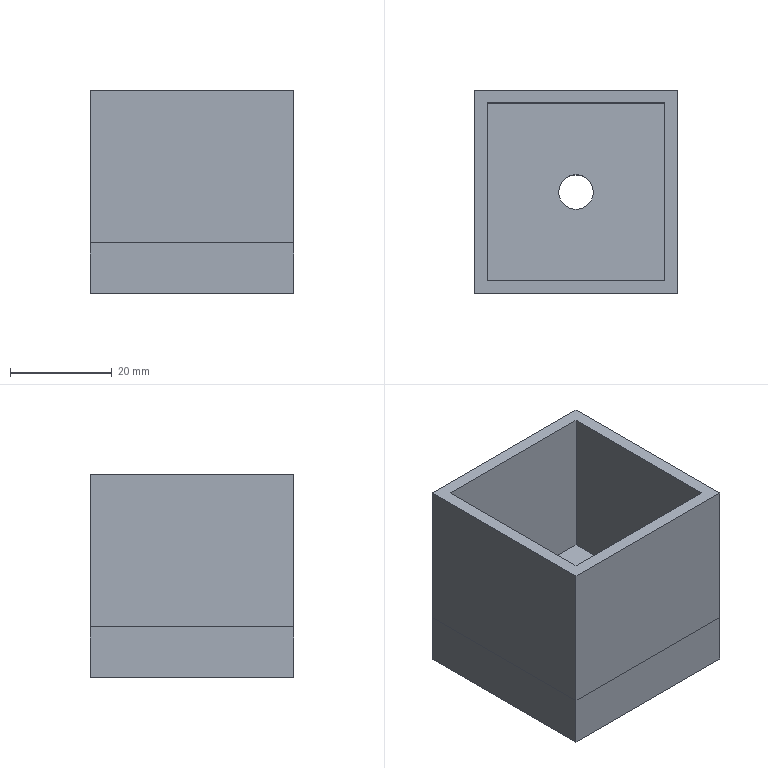Component | SolidWorks | SYM0671-81-101-1_SYM0636-81-109-1 | 2 solids | 18 faces | box 40 x 40 x 40 mm | volume 26887 mm3 | plane 16 | cylinder 2 | commonest cylinder face diameters 6.8 x2 | material AISI 304
build123d program:
from build123d import *

# Parameters (mm, degrees)
SKETCH1_W           = 40
SKETCH1_H           = 40
SKETCH1_W_2         = 35
SKETCH1_H_2         = 35
EXTRUDE_THIN1_DEPTH = 30
SKETCH2_W           = 40
SKETCH2_H           = 40
BOSS_EXTRUDE1_DEPTH = 10


with BuildPart() as part:
    # Sketch1 → Extrude-Thin1 (new body)
    with BuildSketch(Plane.XY):
        Rectangle(SKETCH1_W, SKETCH1_H)
        Rectangle(SKETCH1_W_2, SKETCH1_H_2, mode=Mode.SUBTRACT)
    extrude(amount=EXTRUDE_THIN1_DEPTH)


with BuildPart() as body_2:
    # Sketch2 → Boss-Extrude1 (new body)
    with BuildSketch(Plane(origin=(0, 0, 0), x_dir=(-1, 0, 0), z_dir=(0, 0, -1))):
        Rectangle(SKETCH2_W, SKETCH2_H)
    extrude(amount=BOSS_EXTRUDE1_DEPTH)

    # Sketch3 → M8 Tapped Hole1 (revolve, cut)
    with BuildSketch(Plane(origin=(0, 0, -10), x_dir=(0, 1, 0), z_dir=(1, 0, 0))):
        Polygon((0, 0), (0, 21.793), (3.4, 19.75), (3.4, 0), align=None)
    revolve(axis=Axis((0, 0, -16.35), (0, 0, 1)), mode=Mode.SUBTRACT)


solid = Compound([part.part, body_2.part])

# Placed as in the assembly
solid = solid.moved(Location((-382.749, 43.143, 439.518), (0, 0, 0)))
STEP:
#1=COLOUR_RGB('',0.7922,0.8196,0.9333);
#2=FILL_AREA_STYLE_COLOUR('',#1);
#3=FILL_AREA_STYLE('',(#2));
#4=SURFACE_STYLE_FILL_AREA(#3);
#5=SURFACE_SIDE_STYLE('',(#4));
#6=SURFACE_STYLE_USAGE(.BOTH.,#5);
#7=PRESENTATION_STYLE_ASSIGNMENT((#6));
#8=CARTESIAN_POINT('',(-15.203,1.699,17.304));
#9=VERTEX_POINT('',#8);
#10=CARTESIAN_POINT('',(-14.935,1.699,17.304));
#11=VERTEX_POINT('',#10);
#12=CARTESIAN_POINT('',(-15.069,1.699,17.304));
#13=DIRECTION('',(0.,0.,1.));
#14=DIRECTION('',(1.,0.,0.));
#15=AXIS2_PLACEMENT_3D('',#12,#13,#14);
#16=CIRCLE('',#15,0.1339);
#17=EDGE_CURVE('',#9,#11,#16,.T.);
#18=ORIENTED_EDGE('',*,*,#17,.T.);
#19=CARTESIAN_POINT('',(-14.935,1.699,16.91));
#20=VERTEX_POINT('',#19);
#21=CARTESIAN_POINT('',(-14.935,1.699,16.91));
#22=DIRECTION('',(0.,0.,-1.));
#23=VECTOR('',#22,39.37);
#24=LINE('',#21,#23);
#25=EDGE_CURVE('',#11,#20,#24,.T.);
#26=ORIENTED_EDGE('',*,*,#25,.T.);
#27=CARTESIAN_POINT('',(-15.203,1.699,16.91));
#28=VERTEX_POINT('',#27);
#29=CARTESIAN_POINT('',(-15.069,1.699,16.91));
#30=DIRECTION('',(0.,0.,-1.));
#31=DIRECTION('',(-1.,0.,0.));
#32=AXIS2_PLACEMENT_3D('',#29,#30,#31);
#33=CIRCLE('',#32,0.1339);
#34=EDGE_CURVE('',#20,#28,#33,.T.);
#35=ORIENTED_EDGE('',*,*,#34,.T.);
#36=CARTESIAN_POINT('',(-15.203,1.699,16.91));
#37=DIRECTION('',(0.,0.,-1.));
#38=VECTOR('',#37,39.37);
#39=LINE('',#36,#38);
#40=EDGE_CURVE('',#9,#28,#39,.T.);
#41=ORIENTED_EDGE('',*,*,#40,.F.);
#42=EDGE_LOOP('',(#18,#26,#35,#41));
#43=FACE_OUTER_BOUND('',#42,.T.);
#44=CARTESIAN_POINT('',(-15.069,1.699,16.91));
#45=DIRECTION('',(0.,0.,-1.));
#46=DIRECTION('',(-1.,0.,0.));
#47=AXIS2_PLACEMENT_3D('',#44,#45,#46);
#48=CYLINDRICAL_SURFACE('',#47,0.1339);
#49=ADVANCED_FACE('',(#43),#48,.F.);
#50=CARTESIAN_POINT('',(-15.856,0.9112,17.304));
#51=VERTEX_POINT('',#50);
#52=CARTESIAN_POINT('',(-15.856,2.486,17.304));
#53=VERTEX_POINT('',#52);
#54=CARTESIAN_POINT('',(-15.856,0.9112,17.304));
#55=DIRECTION('',(0.,1.,0.));
#56=VECTOR('',#55,39.37);
#57=LINE('',#54,#56);
#58=EDGE_CURVE('',#51,#53,#57,.T.);
#59=ORIENTED_EDGE('',*,*,#58,.T.);
#60=CARTESIAN_POINT('',(-15.856,2.486,16.91));
#61=VERTEX_POINT('',#60);
#62=CARTESIAN_POINT('',(-15.856,2.486,16.91));
#63=DIRECTION('',(0.,0.,1.));
#64=VECTOR('',#63,39.37);
#65=LINE('',#62,#64);
#66=EDGE_CURVE('',#61,#53,#65,.T.);
#67=ORIENTED_EDGE('',*,*,#66,.F.);
#68=CARTESIAN_POINT('',(-15.856,0.9112,16.91));
#69=VERTEX_POINT('',#68);
#70=CARTESIAN_POINT('',(-15.856,0.9112,16.91));
#71=DIRECTION('',(0.,1.,0.));
#72=VECTOR('',#71,39.37);
#73=LINE('',#70,#72);
#74=EDGE_CURVE('',#69,#61,#73,.T.);
#75=ORIENTED_EDGE('',*,*,#74,.F.);
#76=CARTESIAN_POINT('',(-15.856,0.9112,16.91));
#77=DIRECTION('',(0.,0.,1.));
#78=VECTOR('',#77,39.37);
#79=LINE('',#76,#78);
#80=EDGE_CURVE('',#69,#51,#79,.T.);
#81=ORIENTED_EDGE('',*,*,#80,.T.);
#82=EDGE_LOOP('',(#59,#67,#75,#81));
#83=FACE_OUTER_BOUND('',#82,.T.);
#84=CARTESIAN_POINT('',(-15.856,0.9112,16.91));
#85=DIRECTION('',(1.,0.,0.));
#86=DIRECTION('',(0.,0.,-1.));
#87=AXIS2_PLACEMENT_3D('',#84,#85,#86);
#88=PLANE('',#87);
#89=ADVANCED_FACE('',(#83),#88,.F.);
#90=CARTESIAN_POINT('',(-14.281,2.486,17.304));
#91=VERTEX_POINT('',#90);
#92=CARTESIAN_POINT('',(-14.281,2.486,17.304));
#93=DIRECTION('',(1.,0.,0.));
#94=VECTOR('',#93,39.37);
#95=LINE('',#92,#94);
#96=EDGE_CURVE('',#53,#91,#95,.T.);
#97=ORIENTED_EDGE('',*,*,#96,.T.);
#98=CARTESIAN_POINT('',(-14.281,2.486,16.91));
#99=VERTEX_POINT('',#98);
#100=CARTESIAN_POINT('',(-14.281,2.486,16.91));
#101=DIRECTION('',(0.,0.,1.));
#102=VECTOR('',#101,39.37);
#103=LINE('',#100,#102);
#104=EDGE_CURVE('',#99,#91,#103,.T.);
#105=ORIENTED_EDGE('',*,*,#104,.F.);
#106=CARTESIAN_POINT('',(-14.281,2.486,16.91));
#107=DIRECTION('',(1.,0.,0.));
#108=VECTOR('',#107,39.37);
#109=LINE('',#106,#108);
#110=EDGE_CURVE('',#61,#99,#109,.T.);
#111=ORIENTED_EDGE('',*,*,#110,.F.);
#112=ORIENTED_EDGE('',*,*,#66,.T.);
#113=EDGE_LOOP('',(#97,#105,#111,#112));
#114=FACE_OUTER_BOUND('',#113,.T.);
#115=CARTESIAN_POINT('',(-14.281,2.486,16.91));
#116=DIRECTION('',(0.,-1.,0.));
#117=DIRECTION('',(0.,0.,-1.));
#118=AXIS2_PLACEMENT_3D('',#115,#116,#117);
#119=PLANE('',#118);
#120=ADVANCED_FACE('',(#114),#119,.F.);
#121=CARTESIAN_POINT('',(-14.281,0.9112,17.304));
#122=VERTEX_POINT('',#121);
#123=CARTESIAN_POINT('',(-14.281,0.9112,17.304));
#124=DIRECTION('',(0.,-1.,0.));
#125=VECTOR('',#124,39.37);
#126=LINE('',#123,#125);
#127=EDGE_CURVE('',#91,#122,#126,.T.);
#128=ORIENTED_EDGE('',*,*,#127,.T.);
#129=CARTESIAN_POINT('',(-14.281,0.9112,16.91));
#130=VERTEX_POINT('',#129);
#131=CARTESIAN_POINT('',(-14.281,0.9112,16.91));
#132=DIRECTION('',(0.,0.,1.));
#133=VECTOR('',#132,39.37);
#134=LINE('',#131,#133);
#135=EDGE_CURVE('',#130,#122,#134,.T.);
#136=ORIENTED_EDGE('',*,*,#135,.F.);
#137=CARTESIAN_POINT('',(-14.281,0.9112,16.91));
#138=DIRECTION('',(0.,-1.,0.));
#139=VECTOR('',#138,39.37);
#140=LINE('',#137,#139);
#141=EDGE_CURVE('',#99,#130,#140,.T.);
#142=ORIENTED_EDGE('',*,*,#141,.F.);
#143=ORIENTED_EDGE('',*,*,#104,.T.);
#144=EDGE_LOOP('',(#128,#136,#142,#143));
#145=FACE_OUTER_BOUND('',#144,.T.);
#146=CARTESIAN_POINT('',(-14.281,0.9112,16.91));
#147=DIRECTION('',(-1.,0.,0.));
#148=DIRECTION('',(0.,0.,1.));
#149=AXIS2_PLACEMENT_3D('',#146,#147,#148);
#150=PLANE('',#149);
#151=ADVANCED_FACE('',(#145),#150,.F.);
#152=CARTESIAN_POINT('',(-14.281,0.9112,17.304));
#153=DIRECTION('',(-1.,0.,0.));
#154=VECTOR('',#153,39.37);
#155=LINE('',#152,#154);
#156=EDGE_CURVE('',#122,#51,#155,.T.);
#157=ORIENTED_EDGE('',*,*,#156,.T.);
#158=ORIENTED_EDGE('',*,*,#80,.F.);
#159=CARTESIAN_POINT('',(-14.281,0.9112,16.91));
#160=DIRECTION('',(-1.,0.,0.));
#161=VECTOR('',#160,39.37);
#162=LINE('',#159,#161);
#163=EDGE_CURVE('',#130,#69,#162,.T.);
#164=ORIENTED_EDGE('',*,*,#163,.F.);
#165=ORIENTED_EDGE('',*,*,#135,.T.);
#166=EDGE_LOOP('',(#157,#158,#164,#165));
#167=FACE_OUTER_BOUND('',#166,.T.);
#168=CARTESIAN_POINT('',(-14.281,0.9112,16.91));
#169=DIRECTION('',(0.,1.,0.));
#170=DIRECTION('',(0.,0.,1.));
#171=AXIS2_PLACEMENT_3D('',#168,#169,#170);
#172=PLANE('',#171);
#173=ADVANCED_FACE('',(#167),#172,.F.);
#174=CARTESIAN_POINT('',(-15.069,1.699,16.91));
#175=DIRECTION('',(0.,0.,-1.));
#176=DIRECTION('',(-1.,0.,0.));
#177=AXIS2_PLACEMENT_3D('',#174,#175,#176);
#178=CIRCLE('',#177,0.1339);
#179=EDGE_CURVE('',#28,#20,#178,.T.);
#180=ORIENTED_EDGE('',*,*,#179,.F.);
#181=ORIENTED_EDGE('',*,*,#34,.F.);
#182=EDGE_LOOP('',(#180,#181));
#183=FACE_BOUND('',#182,.T.);
#184=ORIENTED_EDGE('',*,*,#74,.T.);
#185=ORIENTED_EDGE('',*,*,#110,.T.);
#186=ORIENTED_EDGE('',*,*,#141,.T.);
#187=ORIENTED_EDGE('',*,*,#163,.T.);
#188=EDGE_LOOP('',(#184,#185,#186,#187));
#189=FACE_OUTER_BOUND('',#188,.T.);
#190=CARTESIAN_POINT('',(-15.856,2.486,16.91));
#191=DIRECTION('',(0.,0.,1.));
#192=DIRECTION('',(1.,0.,0.));
#193=AXIS2_PLACEMENT_3D('',#190,#191,#192);
#194=PLANE('',#193);
#195=ADVANCED_FACE('',(#183,#189),#194,.F.);
#196=ORIENTED_EDGE('',*,*,#17,.F.);
#197=CARTESIAN_POINT('',(-15.069,1.699,17.304));
#198=DIRECTION('',(0.,0.,1.));
#199=DIRECTION('',(1.,0.,0.));
#200=AXIS2_PLACEMENT_3D('',#197,#198,#199);
#201=CIRCLE('',#200,0.1339);
#202=EDGE_CURVE('',#11,#9,#201,.T.);
#203=ORIENTED_EDGE('',*,*,#202,.F.);
#204=EDGE_LOOP('',(#196,#203));
#205=FACE_BOUND('',#204,.T.);
#206=ORIENTED_EDGE('',*,*,#58,.F.);
#207=ORIENTED_EDGE('',*,*,#156,.F.);
#208=ORIENTED_EDGE('',*,*,#127,.F.);
#209=ORIENTED_EDGE('',*,*,#96,.F.);
#210=EDGE_LOOP('',(#206,#207,#208,#209));
#211=FACE_OUTER_BOUND('',#210,.T.);
#212=CARTESIAN_POINT('',(-15.856,2.486,17.304));
#213=DIRECTION('',(0.,0.,1.));
#214=DIRECTION('',(1.,0.,0.));
#215=AXIS2_PLACEMENT_3D('',#212,#213,#214);
#216=PLANE('',#215);
#217=ADVANCED_FACE('',(#205,#211),#216,.T.);
#218=ORIENTED_EDGE('',*,*,#25,.F.);
#219=ORIENTED_EDGE('',*,*,#202,.T.);
#220=ORIENTED_EDGE('',*,*,#40,.T.);
#221=ORIENTED_EDGE('',*,*,#179,.T.);
#222=EDGE_LOOP('',(#218,#219,#220,#221));
#223=FACE_OUTER_BOUND('',#222,.T.);
#224=CARTESIAN_POINT('',(-15.069,1.699,16.91));
#225=DIRECTION('',(0.,0.,-1.));
#226=DIRECTION('',(-1.,0.,0.));
#227=AXIS2_PLACEMENT_3D('',#224,#225,#226);
#228=CYLINDRICAL_SURFACE('',#227,0.1339);
#229=ADVANCED_FACE('',(#223),#228,.F.);
#230=CLOSED_SHELL('',(#49,#89,#120,#151,#173,#195,#217,#229));
#231=MANIFOLD_SOLID_BREP('',#230);
#232=STYLED_ITEM('',(#7),#231);
#233=(LENGTH_UNIT()NAMED_UNIT(*)SI_UNIT($,.METRE.));
#234=LENGTH_MEASURE_WITH_UNIT(LENGTH_MEASURE(0.0254),#233);
#235=DIMENSIONAL_EXPONENTS(1.,0.,0.,0.,0.,0.,0.);
#236=(CONVERSION_BASED_UNIT('',#234)LENGTH_UNIT()NAMED_UNIT(#235));
#237=UNCERTAINTY_MEASURE_WITH_UNIT(LENGTH_MEASURE(0.00001),#236,'','');
#238=(NAMED_UNIT(*)PLANE_ANGLE_UNIT()SI_UNIT($,.RADIAN.));
#239=(NAMED_UNIT(*)SI_UNIT($,.STERADIAN.)SOLID_ANGLE_UNIT());
#240=(GEOMETRIC_REPRESENTATION_CONTEXT(3)GLOBAL_UNCERTAINTY_ASSIGNED_CONTEXT((#237))GLOBAL_UNIT_ASSIGNED_CONTEXT((#236,#238,#239))REPRESENTATION_CONTEXT('',''));
#241=MECHANICAL_DESIGN_GEOMETRIC_PRESENTATION_REPRESENTATION('',(#232),#240);
#242=COLOUR_RGB('',0.7922,0.8196,0.9333);
#243=FILL_AREA_STYLE_COLOUR('',#242);
#244=FILL_AREA_STYLE('',(#243));
#245=SURFACE_STYLE_FILL_AREA(#244);
#246=SURFACE_SIDE_STYLE('',(#245));
#247=SURFACE_STYLE_USAGE(.BOTH.,#246);
#248=PRESENTATION_STYLE_ASSIGNMENT((#247));
#249=CARTESIAN_POINT('',(-14.281,0.9112,18.485));
#250=VERTEX_POINT('',#249);
#251=CARTESIAN_POINT('',(-14.281,2.486,18.485));
#252=VERTEX_POINT('',#251);
#253=CARTESIAN_POINT('',(-14.281,2.486,18.485));
#254=DIRECTION('',(-0.,1.,0.));
#255=VECTOR('',#254,39.37);
#256=LINE('',#253,#255);
#257=EDGE_CURVE('',#250,#252,#256,.T.);
#258=ORIENTED_EDGE('',*,*,#257,.T.);
#259=CARTESIAN_POINT('',(-15.856,2.486,18.485));
#260=VERTEX_POINT('',#259);
#261=CARTESIAN_POINT('',(-15.856,2.486,18.485));
#262=DIRECTION('',(-1.,0.,0.));
#263=VECTOR('',#262,39.37);
#264=LINE('',#261,#263);
#265=EDGE_CURVE('',#252,#260,#264,.T.);
#266=ORIENTED_EDGE('',*,*,#265,.T.);
#267=CARTESIAN_POINT('',(-15.856,0.9112,18.485));
#268=VERTEX_POINT('',#267);
#269=CARTESIAN_POINT('',(-15.856,2.486,18.485));
#270=DIRECTION('',(0.,-1.,0.));
#271=VECTOR('',#270,39.37);
#272=LINE('',#269,#271);
#273=EDGE_CURVE('',#260,#268,#272,.T.);
#274=ORIENTED_EDGE('',*,*,#273,.T.);
#275=CARTESIAN_POINT('',(-15.856,0.9112,18.485));
#276=DIRECTION('',(1.,0.,0.));
#277=VECTOR('',#276,39.37);
#278=LINE('',#275,#277);
#279=EDGE_CURVE('',#268,#250,#278,.T.);
#280=ORIENTED_EDGE('',*,*,#279,.T.);
#281=EDGE_LOOP('',(#258,#266,#274,#280));
#282=FACE_OUTER_BOUND('',#281,.T.);
#283=CARTESIAN_POINT('',(-14.38,2.388,18.485));
#284=VERTEX_POINT('',#283);
#285=CARTESIAN_POINT('',(-15.758,2.388,18.485));
#286=VERTEX_POINT('',#285);
#287=CARTESIAN_POINT('',(-15.856,2.388,18.485));
#288=DIRECTION('',(-1.,0.,0.));
#289=VECTOR('',#288,39.37);
#290=LINE('',#287,#289);
#291=EDGE_CURVE('',#284,#286,#290,.T.);
#292=ORIENTED_EDGE('',*,*,#291,.F.);
#293=CARTESIAN_POINT('',(-14.38,1.01,18.485));
#294=VERTEX_POINT('',#293);
#295=CARTESIAN_POINT('',(-14.38,2.486,18.485));
#296=DIRECTION('',(-0.,1.,0.));
#297=VECTOR('',#296,39.37);
#298=LINE('',#295,#297);
#299=EDGE_CURVE('',#294,#284,#298,.T.);
#300=ORIENTED_EDGE('',*,*,#299,.F.);
#301=CARTESIAN_POINT('',(-15.758,1.01,18.485));
#302=VERTEX_POINT('',#301);
#303=CARTESIAN_POINT('',(-15.856,1.01,18.485));
#304=DIRECTION('',(1.,0.,0.));
#305=VECTOR('',#304,39.37);
#306=LINE('',#303,#305);
#307=EDGE_CURVE('',#302,#294,#306,.T.);
#308=ORIENTED_EDGE('',*,*,#307,.F.);
#309=CARTESIAN_POINT('',(-15.758,2.486,18.485));
#310=DIRECTION('',(0.,-1.,0.));
#311=VECTOR('',#310,39.37);
#312=LINE('',#309,#311);
#313=EDGE_CURVE('',#286,#302,#312,.T.);
#314=ORIENTED_EDGE('',*,*,#313,.F.);
#315=EDGE_LOOP('',(#292,#300,#308,#314));
#316=FACE_BOUND('',#315,.T.);
#317=CARTESIAN_POINT('',(-14.281,2.486,18.485));
#318=DIRECTION('',(0.,0.,1.));
#319=DIRECTION('',(1.,0.,0.));
#320=AXIS2_PLACEMENT_3D('',#317,#318,#319);
#321=PLANE('',#320);
#322=ADVANCED_FACE('',(#282,#316),#321,.T.);
#323=CARTESIAN_POINT('',(-14.281,0.9112,17.304));
#324=VERTEX_POINT('',#323);
#325=CARTESIAN_POINT('',(-14.281,2.486,17.304));
#326=VERTEX_POINT('',#325);
#327=CARTESIAN_POINT('',(-14.281,2.486,17.304));
#328=DIRECTION('',(-0.,1.,0.));
#329=VECTOR('',#328,39.37);
#330=LINE('',#327,#329);
#331=EDGE_CURVE('',#324,#326,#330,.T.);
#332=ORIENTED_EDGE('',*,*,#331,.F.);
#333=CARTESIAN_POINT('',(-15.856,0.9112,17.304));
#334=VERTEX_POINT('',#333);
#335=CARTESIAN_POINT('',(-15.856,0.9112,17.304));
#336=DIRECTION('',(1.,0.,0.));
#337=VECTOR('',#336,39.37);
#338=LINE('',#335,#337);
#339=EDGE_CURVE('',#334,#324,#338,.T.);
#340=ORIENTED_EDGE('',*,*,#339,.F.);
#341=CARTESIAN_POINT('',(-15.856,2.486,17.304));
#342=VERTEX_POINT('',#341);
#343=CARTESIAN_POINT('',(-15.856,2.486,17.304));
#344=DIRECTION('',(0.,-1.,0.));
#345=VECTOR('',#344,39.37);
#346=LINE('',#343,#345);
#347=EDGE_CURVE('',#342,#334,#346,.T.);
#348=ORIENTED_EDGE('',*,*,#347,.F.);
#349=CARTESIAN_POINT('',(-15.856,2.486,17.304));
#350=DIRECTION('',(-1.,0.,0.));
#351=VECTOR('',#350,39.37);
#352=LINE('',#349,#351);
#353=EDGE_CURVE('',#326,#342,#352,.T.);
#354=ORIENTED_EDGE('',*,*,#353,.F.);
#355=EDGE_LOOP('',(#332,#340,#348,#354));
#356=FACE_OUTER_BOUND('',#355,.T.);
#357=CARTESIAN_POINT('',(-14.38,1.01,17.304));
#358=VERTEX_POINT('',#357);
#359=CARTESIAN_POINT('',(-14.38,2.388,17.304));
#360=VERTEX_POINT('',#359);
#361=CARTESIAN_POINT('',(-14.38,2.486,17.304));
#362=DIRECTION('',(-0.,1.,0.));
#363=VECTOR('',#362,39.37);
#364=LINE('',#361,#363);
#365=EDGE_CURVE('',#358,#360,#364,.T.);
#366=ORIENTED_EDGE('',*,*,#365,.T.);
#367=CARTESIAN_POINT('',(-15.758,2.388,17.304));
#368=VERTEX_POINT('',#367);
#369=CARTESIAN_POINT('',(-15.856,2.388,17.304));
#370=DIRECTION('',(-1.,0.,0.));
#371=VECTOR('',#370,39.37);
#372=LINE('',#369,#371);
#373=EDGE_CURVE('',#360,#368,#372,.T.);
#374=ORIENTED_EDGE('',*,*,#373,.T.);
#375=CARTESIAN_POINT('',(-15.758,1.01,17.304));
#376=VERTEX_POINT('',#375);
#377=CARTESIAN_POINT('',(-15.758,2.486,17.304));
#378=DIRECTION('',(0.,-1.,0.));
#379=VECTOR('',#378,39.37);
#380=LINE('',#377,#379);
#381=EDGE_CURVE('',#368,#376,#380,.T.);
#382=ORIENTED_EDGE('',*,*,#381,.T.);
#383=CARTESIAN_POINT('',(-15.856,1.01,17.304));
#384=DIRECTION('',(1.,0.,0.));
#385=VECTOR('',#384,39.37);
#386=LINE('',#383,#385);
#387=EDGE_CURVE('',#376,#358,#386,.T.);
#388=ORIENTED_EDGE('',*,*,#387,.T.);
#389=EDGE_LOOP('',(#366,#374,#382,#388));
#390=FACE_BOUND('',#389,.T.);
#391=CARTESIAN_POINT('',(-14.281,2.486,17.304));
#392=DIRECTION('',(0.,0.,1.));
#393=DIRECTION('',(1.,0.,0.));
#394=AXIS2_PLACEMENT_3D('',#391,#392,#393);
#395=PLANE('',#394);
#396=ADVANCED_FACE('',(#356,#390),#395,.F.);
#397=ORIENTED_EDGE('',*,*,#331,.T.);
#398=CARTESIAN_POINT('',(-14.281,2.486,18.485));
#399=DIRECTION('',(0.,0.,-1.));
#400=VECTOR('',#399,39.37);
#401=LINE('',#398,#400);
#402=EDGE_CURVE('',#252,#326,#401,.T.);
#403=ORIENTED_EDGE('',*,*,#402,.F.);
#404=ORIENTED_EDGE('',*,*,#257,.F.);
#405=CARTESIAN_POINT('',(-14.281,0.9112,18.485));
#406=DIRECTION('',(0.,0.,-1.));
#407=VECTOR('',#406,39.37);
#408=LINE('',#405,#407);
#409=EDGE_CURVE('',#250,#324,#408,.T.);
#410=ORIENTED_EDGE('',*,*,#409,.T.);
#411=EDGE_LOOP('',(#397,#403,#404,#410));
#412=FACE_OUTER_BOUND('',#411,.T.);
#413=CARTESIAN_POINT('',(-14.281,2.486,18.485));
#414=DIRECTION('',(-1.,-0.,0.));
#415=DIRECTION('',(0.,-1.,0.));
#416=AXIS2_PLACEMENT_3D('',#413,#414,#415);
#417=PLANE('',#416);
#418=ADVANCED_FACE('',(#412),#417,.F.);
#419=ORIENTED_EDGE('',*,*,#353,.T.);
#420=CARTESIAN_POINT('',(-15.856,2.486,18.485));
#421=DIRECTION('',(0.,0.,-1.));
#422=VECTOR('',#421,39.37);
#423=LINE('',#420,#422);
#424=EDGE_CURVE('',#260,#342,#423,.T.);
#425=ORIENTED_EDGE('',*,*,#424,.F.);
#426=ORIENTED_EDGE('',*,*,#265,.F.);
#427=ORIENTED_EDGE('',*,*,#402,.T.);
#428=EDGE_LOOP('',(#419,#425,#426,#427));
#429=FACE_OUTER_BOUND('',#428,.T.);
#430=CARTESIAN_POINT('',(-15.856,2.486,18.485));
#431=DIRECTION('',(0.,-1.,0.));
#432=DIRECTION('',(0.,0.,-1.));
#433=AXIS2_PLACEMENT_3D('',#430,#431,#432);
#434=PLANE('',#433);
#435=ADVANCED_FACE('',(#429),#434,.F.);
#436=ORIENTED_EDGE('',*,*,#347,.T.);
#437=CARTESIAN_POINT('',(-15.856,0.9112,18.485));
#438=DIRECTION('',(0.,0.,-1.));
#439=VECTOR('',#438,39.37);
#440=LINE('',#437,#439);
#441=EDGE_CURVE('',#268,#334,#440,.T.);
#442=ORIENTED_EDGE('',*,*,#441,.F.);
#443=ORIENTED_EDGE('',*,*,#273,.F.);
#444=ORIENTED_EDGE('',*,*,#424,.T.);
#445=EDGE_LOOP('',(#436,#442,#443,#444));
#446=FACE_OUTER_BOUND('',#445,.T.);
#447=CARTESIAN_POINT('',(-15.856,2.486,18.485));
#448=DIRECTION('',(1.,0.,0.));
#449=DIRECTION('',(-0.,1.,0.));
#450=AXIS2_PLACEMENT_3D('',#447,#448,#449);
#451=PLANE('',#450);
#452=ADVANCED_FACE('',(#446),#451,.F.);
#453=ORIENTED_EDGE('',*,*,#339,.T.);
#454=ORIENTED_EDGE('',*,*,#409,.F.);
#455=ORIENTED_EDGE('',*,*,#279,.F.);
#456=ORIENTED_EDGE('',*,*,#441,.T.);
#457=EDGE_LOOP('',(#453,#454,#455,#456));
#458=FACE_OUTER_BOUND('',#457,.T.);
#459=CARTESIAN_POINT('',(-15.856,0.9112,18.485));
#460=DIRECTION('',(0.,1.,0.));
#461=DIRECTION('',(0.,0.,1.));
#462=AXIS2_PLACEMENT_3D('',#459,#460,#461);
#463=PLANE('',#462);
#464=ADVANCED_FACE('',(#458),#463,.F.);
#465=ORIENTED_EDGE('',*,*,#365,.F.);
#466=CARTESIAN_POINT('',(-14.38,1.01,18.485));
#467=DIRECTION('',(0.,0.,-1.));
#468=VECTOR('',#467,39.37);
#469=LINE('',#466,#468);
#470=EDGE_CURVE('',#294,#358,#469,.T.);
#471=ORIENTED_EDGE('',*,*,#470,.F.);
#472=ORIENTED_EDGE('',*,*,#299,.T.);
#473=CARTESIAN_POINT('',(-14.38,2.388,18.485));
#474=DIRECTION('',(0.,0.,-1.));
#475=VECTOR('',#474,39.37);
#476=LINE('',#473,#475);
#477=EDGE_CURVE('',#284,#360,#476,.T.);
#478=ORIENTED_EDGE('',*,*,#477,.T.);
#479=EDGE_LOOP('',(#465,#471,#472,#478));
#480=FACE_OUTER_BOUND('',#479,.T.);
#481=CARTESIAN_POINT('',(-14.38,2.486,18.485));
#482=DIRECTION('',(-1.,-0.,0.));
#483=DIRECTION('',(0.,-1.,0.));
#484=AXIS2_PLACEMENT_3D('',#481,#482,#483);
#485=PLANE('',#484);
#486=ADVANCED_FACE('',(#480),#485,.T.);
#487=ORIENTED_EDGE('',*,*,#373,.F.);
#488=ORIENTED_EDGE('',*,*,#477,.F.);
#489=ORIENTED_EDGE('',*,*,#291,.T.);
#490=CARTESIAN_POINT('',(-15.758,2.388,18.485));
#491=DIRECTION('',(0.,0.,-1.));
#492=VECTOR('',#491,39.37);
#493=LINE('',#490,#492);
#494=EDGE_CURVE('',#286,#368,#493,.T.);
#495=ORIENTED_EDGE('',*,*,#494,.T.);
#496=EDGE_LOOP('',(#487,#488,#489,#495));
#497=FACE_OUTER_BOUND('',#496,.T.);
#498=CARTESIAN_POINT('',(-15.856,2.388,18.485));
#499=DIRECTION('',(0.,-1.,0.));
#500=DIRECTION('',(0.,0.,-1.));
#501=AXIS2_PLACEMENT_3D('',#498,#499,#500);
#502=PLANE('',#501);
#503=ADVANCED_FACE('',(#497),#502,.T.);
#504=ORIENTED_EDGE('',*,*,#381,.F.);
#505=ORIENTED_EDGE('',*,*,#494,.F.);
#506=ORIENTED_EDGE('',*,*,#313,.T.);
#507=CARTESIAN_POINT('',(-15.758,1.01,18.485));
#508=DIRECTION('',(0.,0.,-1.));
#509=VECTOR('',#508,39.37);
#510=LINE('',#507,#509);
#511=EDGE_CURVE('',#302,#376,#510,.T.);
#512=ORIENTED_EDGE('',*,*,#511,.T.);
#513=EDGE_LOOP('',(#504,#505,#506,#512));
#514=FACE_OUTER_BOUND('',#513,.T.);
#515=CARTESIAN_POINT('',(-15.758,2.486,18.485));
#516=DIRECTION('',(1.,0.,0.));
#517=DIRECTION('',(-0.,1.,0.));
#518=AXIS2_PLACEMENT_3D('',#515,#516,#517);
#519=PLANE('',#518);
#520=ADVANCED_FACE('',(#514),#519,.T.);
#521=ORIENTED_EDGE('',*,*,#387,.F.);
#522=ORIENTED_EDGE('',*,*,#511,.F.);
#523=ORIENTED_EDGE('',*,*,#307,.T.);
#524=ORIENTED_EDGE('',*,*,#470,.T.);
#525=EDGE_LOOP('',(#521,#522,#523,#524));
#526=FACE_OUTER_BOUND('',#525,.T.);
#527=CARTESIAN_POINT('',(-15.856,1.01,18.485));
#528=DIRECTION('',(0.,1.,0.));
#529=DIRECTION('',(0.,0.,1.));
#530=AXIS2_PLACEMENT_3D('',#527,#528,#529);
#531=PLANE('',#530);
#532=ADVANCED_FACE('',(#526),#531,.T.);
#533=CLOSED_SHELL('',(#322,#396,#418,#435,#452,#464,#486,#503,#520,#532));
#534=MANIFOLD_SOLID_BREP('',#533);
#535=STYLED_ITEM('',(#248),#534);
#536=(LENGTH_UNIT()NAMED_UNIT(*)SI_UNIT($,.METRE.));
#537=LENGTH_MEASURE_WITH_UNIT(LENGTH_MEASURE(0.0254),#536);
#538=DIMENSIONAL_EXPONENTS(1.,0.,0.,0.,0.,0.,0.);
#539=(CONVERSION_BASED_UNIT('',#537)LENGTH_UNIT()NAMED_UNIT(#538));
#540=UNCERTAINTY_MEASURE_WITH_UNIT(LENGTH_MEASURE(0.00001),#539,'','');
#541=(NAMED_UNIT(*)PLANE_ANGLE_UNIT()SI_UNIT($,.RADIAN.));
#542=(NAMED_UNIT(*)SI_UNIT($,.STERADIAN.)SOLID_ANGLE_UNIT());
#543=(GEOMETRIC_REPRESENTATION_CONTEXT(3)GLOBAL_UNCERTAINTY_ASSIGNED_CONTEXT((#540))GLOBAL_UNIT_ASSIGNED_CONTEXT((#539,#541,#542))REPRESENTATION_CONTEXT('',''));
#544=MECHANICAL_DESIGN_GEOMETRIC_PRESENTATION_REPRESENTATION('',(#535),#543);
#545=PRESENTATION_LAYER_ASSIGNMENT('','',(#232));
#546=CARTESIAN_POINT('',(0.,0.,0.));
#547=DIRECTION('',(0.,0.,1.));
#548=DIRECTION('',(1.,0.,0.));
#549=AXIS2_PLACEMENT_3D('',#546,#547,#548);
#550=(LENGTH_UNIT()NAMED_UNIT(*)SI_UNIT($,.METRE.));
#551=LENGTH_MEASURE_WITH_UNIT(LENGTH_MEASURE(0.0254),#550);
#552=DIMENSIONAL_EXPONENTS(1.,0.,0.,0.,0.,0.,0.);
#553=(CONVERSION_BASED_UNIT('',#551)LENGTH_UNIT()NAMED_UNIT(#552));
#554=UNCERTAINTY_MEASURE_WITH_UNIT(LENGTH_MEASURE(0.00001),#553,'','');
#555=(NAMED_UNIT(*)PLANE_ANGLE_UNIT()SI_UNIT($,.RADIAN.));
#556=(NAMED_UNIT(*)SI_UNIT($,.STERADIAN.)SOLID_ANGLE_UNIT());
#557=(GEOMETRIC_REPRESENTATION_CONTEXT(3)GLOBAL_UNCERTAINTY_ASSIGNED_CONTEXT((#554))GLOBAL_UNIT_ASSIGNED_CONTEXT((#553,#555,#556))REPRESENTATION_CONTEXT('',''));
#558=ADVANCED_BREP_SHAPE_REPRESENTATION('',(#231,#534,#549),#557);
#559=PRESENTATION_LAYER_ASSIGNMENT('','',(#535));